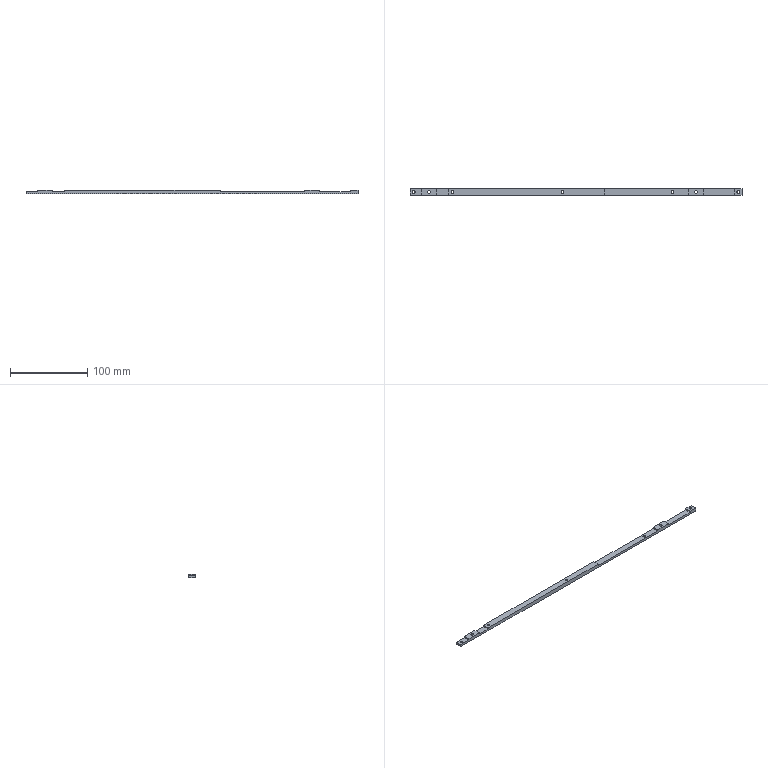CAM job | Mastercam | mm | 6 operations | part box 433.19 x 29.63 x 5
1. Facing | 9 - 10 平铣刀
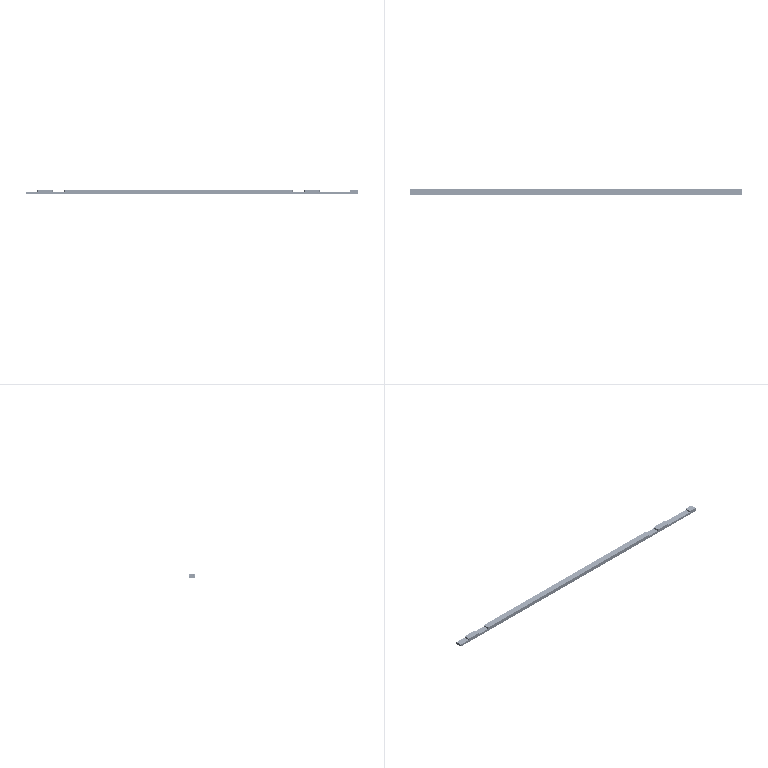2. Contour (2D) | 9 - 10 平铣刀
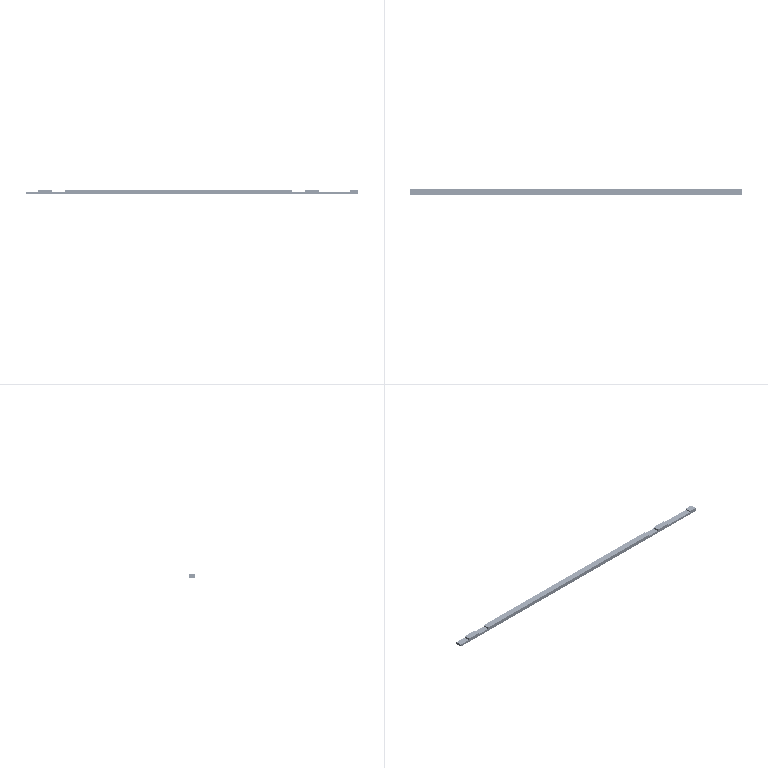3. Drill/Counterbore | 12 - 6 定位钻
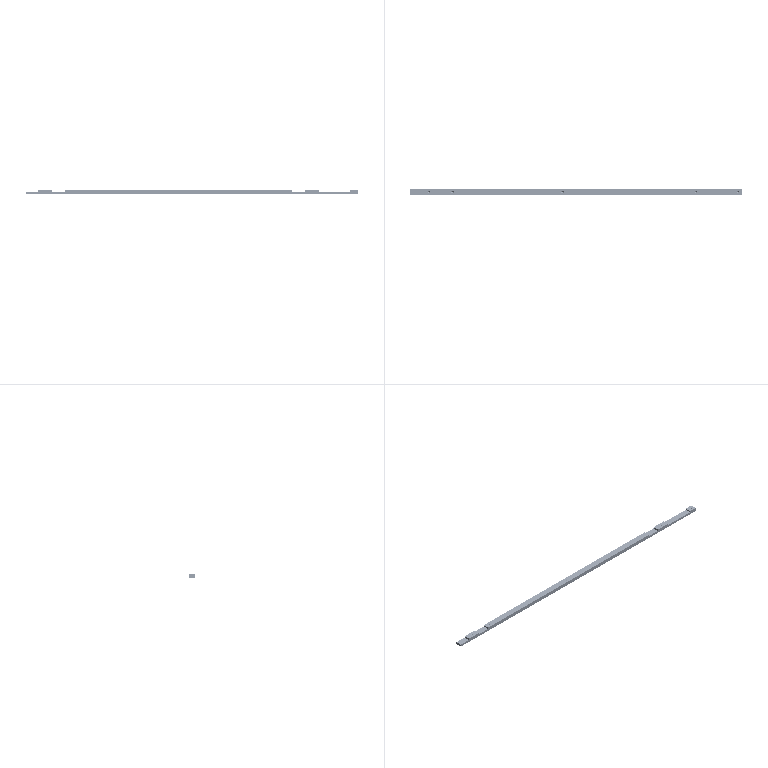4. Drill/Counterbore | 12 - 6 定位钻
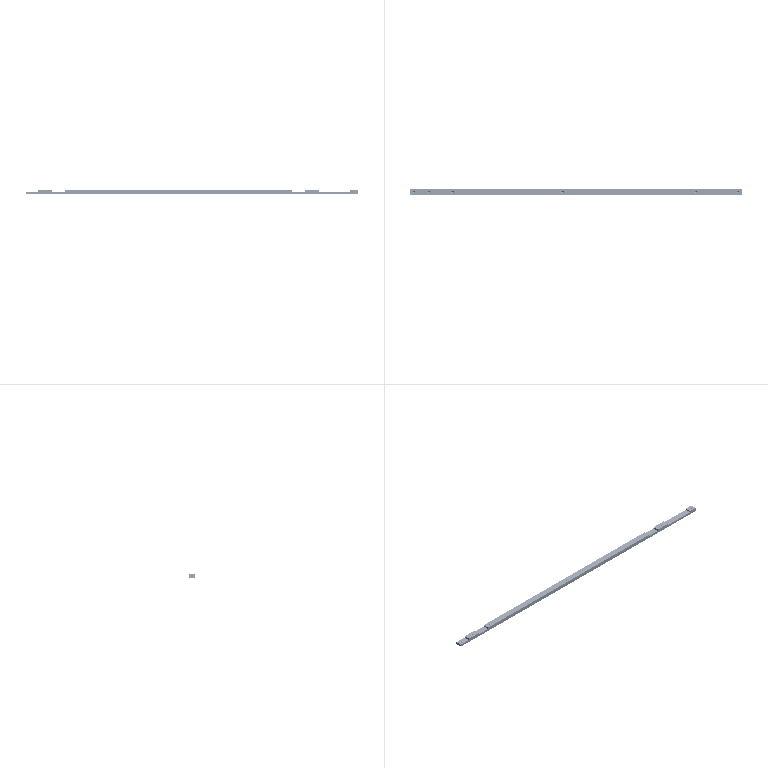5. Drill/Counterbore | 12 - 6 定位钻
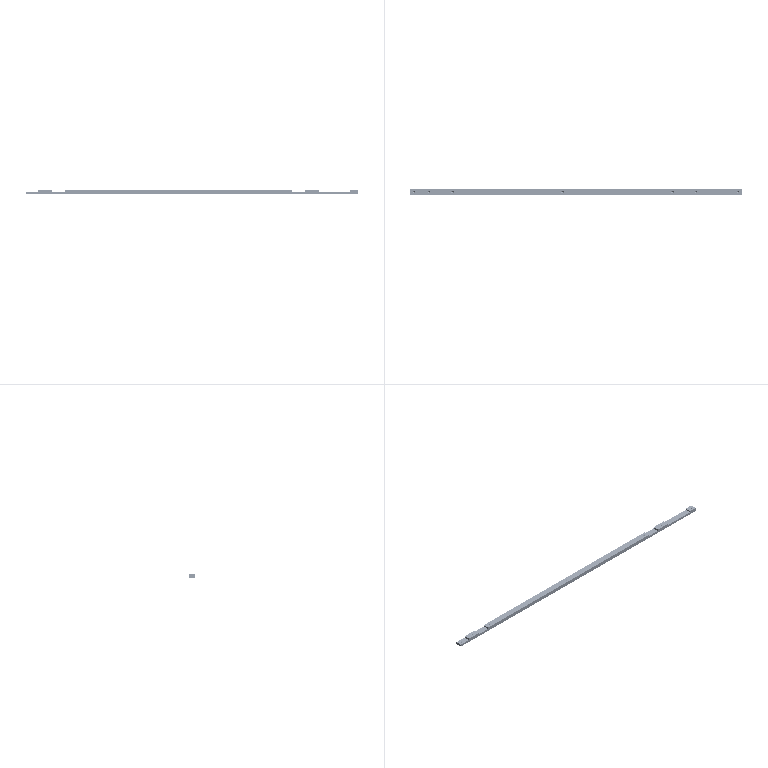6. Peck Drill | 11 - 3.5 钻头